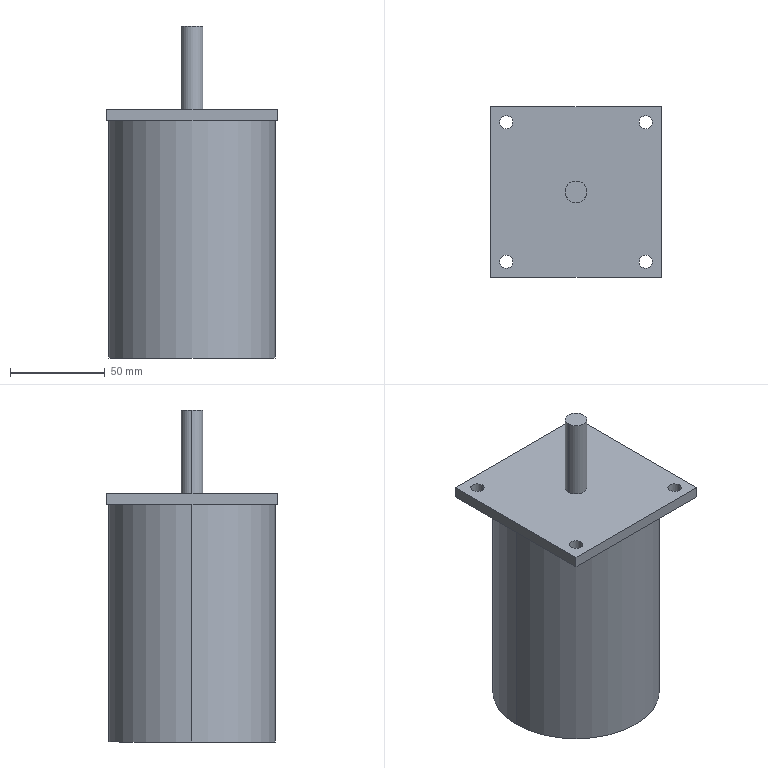Component | SolidWorks | Motor-1 | 1 solid | 20 faces | box 90 x 90 x 175 mm | volume 812512 mm3 | cylinder 12 | plane 8 | commonest cylinder face diameters 7 x8 11.5 x2 88 x2
build123d program:
from build123d import *

# Parameters (mm, degrees)
SKETCH1_W      = 90
SKETCH1_H      = 90
SKETCH1_R      = 3.5
EXTRUDE1_DEPTH = 6
SKETCH2_R      = 44
EXTRUDE2_DEPTH = 125
SKETCH3_R      = 5.75
EXTRUDE3_DEPTH = 44


with BuildPart() as part:
    # Sketch1 → Extrude1 (new body)
    with BuildSketch(Plane.XY):
        Rectangle(SKETCH1_W, SKETCH1_H)
        with Locations((-36.75, 36.75)):
            Circle(SKETCH1_R, mode=Mode.SUBTRACT)
        with Locations((36.75, 36.75)):
            Circle(SKETCH1_R, mode=Mode.SUBTRACT)
        with Locations((36.75, -36.75)):
            Circle(SKETCH1_R, mode=Mode.SUBTRACT)
        with Locations((-36.75, -36.75)):
            Circle(SKETCH1_R, mode=Mode.SUBTRACT)
    extrude(amount=EXTRUDE1_DEPTH)

    # Sketch2 → Extrude2 (add)
    with BuildSketch(Plane.XY.offset(6)):
        Circle(SKETCH2_R)
    extrude(amount=EXTRUDE2_DEPTH)

    # Sketch3 → Extrude3 (add)
    with BuildSketch(Plane(origin=(0, 0, 0), x_dir=(-1, 0, 0), z_dir=(0, 0, -1))):
        with Locations(Location((0, 0, 0), (0, 0, 180))):
            Circle(SKETCH3_R)
    extrude(amount=EXTRUDE3_DEPTH)


solid = part.part

# Placed as in the assembly
solid = solid.moved(Location((-160.944, 693.983, 237.789), (180, 0, 0)))
STEP:
#1=COLOUR_RGB('',0.7922,0.8196,0.9333);
#2=FILL_AREA_STYLE_COLOUR('',#1);
#3=FILL_AREA_STYLE('',(#2));
#4=SURFACE_STYLE_FILL_AREA(#3);
#5=SURFACE_SIDE_STYLE('',(#4));
#6=SURFACE_STYLE_USAGE(.BOTH.,#5);
#7=PRESENTATION_STYLE_ASSIGNMENT((#6));
#8=CARTESIAN_POINT('',(-6.11,27.322,11.094));
#9=VERTEX_POINT('',#8);
#10=CARTESIAN_POINT('',(-6.563,27.322,11.094));
#11=VERTEX_POINT('',#10);
#12=CARTESIAN_POINT('',(-6.336,27.322,11.094));
#13=DIRECTION('',(-0.,-0.,1.));
#14=DIRECTION('',(1.,0.,0.));
#15=AXIS2_PLACEMENT_3D('',#12,#13,#14);
#16=CIRCLE('',#15,0.2264);
#17=EDGE_CURVE('',#9,#11,#16,.T.);
#18=ORIENTED_EDGE('',*,*,#17,.F.);
#19=CARTESIAN_POINT('',(-6.11,27.322,9.362));
#20=VERTEX_POINT('',#19);
#21=CARTESIAN_POINT('',(-6.11,27.322,11.094));
#22=DIRECTION('',(0.,0.,-1.));
#23=VECTOR('',#22,39.37);
#24=LINE('',#21,#23);
#25=EDGE_CURVE('',#9,#20,#24,.T.);
#26=ORIENTED_EDGE('',*,*,#25,.T.);
#27=CARTESIAN_POINT('',(-6.563,27.322,9.362));
#28=VERTEX_POINT('',#27);
#29=CARTESIAN_POINT('',(-6.336,27.322,9.362));
#30=DIRECTION('',(-0.,-0.,1.));
#31=DIRECTION('',(-1.,0.,0.));
#32=AXIS2_PLACEMENT_3D('',#29,#30,#31);
#33=CIRCLE('',#32,0.2264);
#34=EDGE_CURVE('',#20,#28,#33,.T.);
#35=ORIENTED_EDGE('',*,*,#34,.T.);
#36=CARTESIAN_POINT('',(-6.563,27.322,11.094));
#37=DIRECTION('',(0.,0.,-1.));
#38=VECTOR('',#37,39.37);
#39=LINE('',#36,#38);
#40=EDGE_CURVE('',#11,#28,#39,.T.);
#41=ORIENTED_EDGE('',*,*,#40,.F.);
#42=EDGE_LOOP('',(#18,#26,#35,#41));
#43=FACE_OUTER_BOUND('',#42,.T.);
#44=CARTESIAN_POINT('',(-6.336,27.322,11.094));
#45=DIRECTION('',(0.,0.,-1.));
#46=DIRECTION('',(-1.,0.,0.));
#47=AXIS2_PLACEMENT_3D('',#44,#45,#46);
#48=CYLINDRICAL_SURFACE('',#47,0.2264);
#49=ADVANCED_FACE('',(#43),#48,.T.);
#50=CARTESIAN_POINT('',(-8.069,27.322,4.204));
#51=VERTEX_POINT('',#50);
#52=CARTESIAN_POINT('',(-4.604,27.322,4.204));
#53=VERTEX_POINT('',#52);
#54=CARTESIAN_POINT('',(-6.336,27.322,4.204));
#55=DIRECTION('',(0.,0.,-1.));
#56=DIRECTION('',(-1.,0.,0.));
#57=AXIS2_PLACEMENT_3D('',#54,#55,#56);
#58=CIRCLE('',#57,1.732);
#59=EDGE_CURVE('',#51,#53,#58,.T.);
#60=ORIENTED_EDGE('',*,*,#59,.F.);
#61=CARTESIAN_POINT('',(-8.069,27.322,9.126));
#62=VERTEX_POINT('',#61);
#63=CARTESIAN_POINT('',(-8.069,27.322,4.204));
#64=DIRECTION('',(-0.,-0.,1.));
#65=VECTOR('',#64,39.37);
#66=LINE('',#63,#65);
#67=EDGE_CURVE('',#51,#62,#66,.T.);
#68=ORIENTED_EDGE('',*,*,#67,.T.);
#69=CARTESIAN_POINT('',(-4.604,27.322,9.126));
#70=VERTEX_POINT('',#69);
#71=CARTESIAN_POINT('',(-6.336,27.322,9.126));
#72=DIRECTION('',(0.,0.,-1.));
#73=DIRECTION('',(-1.,0.,0.));
#74=AXIS2_PLACEMENT_3D('',#71,#72,#73);
#75=CIRCLE('',#74,1.732);
#76=EDGE_CURVE('',#62,#70,#75,.T.);
#77=ORIENTED_EDGE('',*,*,#76,.T.);
#78=CARTESIAN_POINT('',(-4.604,27.322,4.204));
#79=DIRECTION('',(-0.,-0.,1.));
#80=VECTOR('',#79,39.37);
#81=LINE('',#78,#80);
#82=EDGE_CURVE('',#53,#70,#81,.T.);
#83=ORIENTED_EDGE('',*,*,#82,.F.);
#84=EDGE_LOOP('',(#60,#68,#77,#83));
#85=FACE_OUTER_BOUND('',#84,.T.);
#86=CARTESIAN_POINT('',(-6.336,27.322,4.204));
#87=DIRECTION('',(-0.,-0.,1.));
#88=DIRECTION('',(1.,0.,0.));
#89=AXIS2_PLACEMENT_3D('',#86,#87,#88);
#90=CYLINDRICAL_SURFACE('',#89,1.732);
#91=ADVANCED_FACE('',(#85),#90,.T.);
#92=CARTESIAN_POINT('',(-4.752,25.875,9.126));
#93=VERTEX_POINT('',#92);
#94=CARTESIAN_POINT('',(-5.027,25.875,9.126));
#95=VERTEX_POINT('',#94);
#96=CARTESIAN_POINT('',(-4.89,25.875,9.126));
#97=DIRECTION('',(0.,0.,-1.));
#98=DIRECTION('',(-1.,0.,0.));
#99=AXIS2_PLACEMENT_3D('',#96,#97,#98);
#100=CIRCLE('',#99,0.1378);
#101=EDGE_CURVE('',#93,#95,#100,.T.);
#102=ORIENTED_EDGE('',*,*,#101,.T.);
#103=CARTESIAN_POINT('',(-5.027,25.875,9.362));
#104=VERTEX_POINT('',#103);
#105=CARTESIAN_POINT('',(-5.027,25.875,9.126));
#106=DIRECTION('',(-0.,-0.,1.));
#107=VECTOR('',#106,39.37);
#108=LINE('',#105,#107);
#109=EDGE_CURVE('',#95,#104,#108,.T.);
#110=ORIENTED_EDGE('',*,*,#109,.T.);
#111=CARTESIAN_POINT('',(-4.752,25.875,9.362));
#112=VERTEX_POINT('',#111);
#113=CARTESIAN_POINT('',(-4.89,25.875,9.362));
#114=DIRECTION('',(0.,0.,-1.));
#115=DIRECTION('',(-1.,0.,0.));
#116=AXIS2_PLACEMENT_3D('',#113,#114,#115);
#117=CIRCLE('',#116,0.1378);
#118=EDGE_CURVE('',#112,#104,#117,.T.);
#119=ORIENTED_EDGE('',*,*,#118,.F.);
#120=CARTESIAN_POINT('',(-4.752,25.875,9.126));
#121=DIRECTION('',(-0.,-0.,1.));
#122=VECTOR('',#121,39.37);
#123=LINE('',#120,#122);
#124=EDGE_CURVE('',#93,#112,#123,.T.);
#125=ORIENTED_EDGE('',*,*,#124,.F.);
#126=EDGE_LOOP('',(#102,#110,#119,#125));
#127=FACE_OUTER_BOUND('',#126,.T.);
#128=CARTESIAN_POINT('',(-4.89,25.875,9.126));
#129=DIRECTION('',(-0.,-0.,1.));
#130=DIRECTION('',(1.,0.,0.));
#131=AXIS2_PLACEMENT_3D('',#128,#129,#130);
#132=CYLINDRICAL_SURFACE('',#131,0.1378);
#133=ADVANCED_FACE('',(#127),#132,.F.);
#134=CARTESIAN_POINT('',(-7.645,25.875,9.126));
#135=VERTEX_POINT('',#134);
#136=CARTESIAN_POINT('',(-7.921,25.875,9.126));
#137=VERTEX_POINT('',#136);
#138=CARTESIAN_POINT('',(-7.783,25.875,9.126));
#139=DIRECTION('',(0.,0.,-1.));
#140=DIRECTION('',(-1.,0.,0.));
#141=AXIS2_PLACEMENT_3D('',#138,#139,#140);
#142=CIRCLE('',#141,0.1378);
#143=EDGE_CURVE('',#135,#137,#142,.T.);
#144=ORIENTED_EDGE('',*,*,#143,.T.);
#145=CARTESIAN_POINT('',(-7.921,25.875,9.362));
#146=VERTEX_POINT('',#145);
#147=CARTESIAN_POINT('',(-7.921,25.875,9.126));
#148=DIRECTION('',(-0.,-0.,1.));
#149=VECTOR('',#148,39.37);
#150=LINE('',#147,#149);
#151=EDGE_CURVE('',#137,#146,#150,.T.);
#152=ORIENTED_EDGE('',*,*,#151,.T.);
#153=CARTESIAN_POINT('',(-7.645,25.875,9.362));
#154=VERTEX_POINT('',#153);
#155=CARTESIAN_POINT('',(-7.783,25.875,9.362));
#156=DIRECTION('',(0.,0.,-1.));
#157=DIRECTION('',(-1.,0.,0.));
#158=AXIS2_PLACEMENT_3D('',#155,#156,#157);
#159=CIRCLE('',#158,0.1378);
#160=EDGE_CURVE('',#154,#146,#159,.T.);
#161=ORIENTED_EDGE('',*,*,#160,.F.);
#162=CARTESIAN_POINT('',(-7.645,25.875,9.126));
#163=DIRECTION('',(-0.,-0.,1.));
#164=VECTOR('',#163,39.37);
#165=LINE('',#162,#164);
#166=EDGE_CURVE('',#135,#154,#165,.T.);
#167=ORIENTED_EDGE('',*,*,#166,.F.);
#168=EDGE_LOOP('',(#144,#152,#161,#167));
#169=FACE_OUTER_BOUND('',#168,.T.);
#170=CARTESIAN_POINT('',(-7.783,25.875,9.126));
#171=DIRECTION('',(-0.,-0.,1.));
#172=DIRECTION('',(1.,0.,0.));
#173=AXIS2_PLACEMENT_3D('',#170,#171,#172);
#174=CYLINDRICAL_SURFACE('',#173,0.1378);
#175=ADVANCED_FACE('',(#169),#174,.F.);
#176=CARTESIAN_POINT('',(-7.645,28.769,9.126));
#177=VERTEX_POINT('',#176);
#178=CARTESIAN_POINT('',(-7.921,28.769,9.126));
#179=VERTEX_POINT('',#178);
#180=CARTESIAN_POINT('',(-7.783,28.769,9.126));
#181=DIRECTION('',(0.,0.,-1.));
#182=DIRECTION('',(-1.,0.,0.));
#183=AXIS2_PLACEMENT_3D('',#180,#181,#182);
#184=CIRCLE('',#183,0.1378);
#185=EDGE_CURVE('',#177,#179,#184,.T.);
#186=ORIENTED_EDGE('',*,*,#185,.T.);
#187=CARTESIAN_POINT('',(-7.921,28.769,9.362));
#188=VERTEX_POINT('',#187);
#189=CARTESIAN_POINT('',(-7.921,28.769,9.126));
#190=DIRECTION('',(-0.,-0.,1.));
#191=VECTOR('',#190,39.37);
#192=LINE('',#189,#191);
#193=EDGE_CURVE('',#179,#188,#192,.T.);
#194=ORIENTED_EDGE('',*,*,#193,.T.);
#195=CARTESIAN_POINT('',(-7.645,28.769,9.362));
#196=VERTEX_POINT('',#195);
#197=CARTESIAN_POINT('',(-7.783,28.769,9.362));
#198=DIRECTION('',(0.,0.,-1.));
#199=DIRECTION('',(-1.,0.,0.));
#200=AXIS2_PLACEMENT_3D('',#197,#198,#199);
#201=CIRCLE('',#200,0.1378);
#202=EDGE_CURVE('',#196,#188,#201,.T.);
#203=ORIENTED_EDGE('',*,*,#202,.F.);
#204=CARTESIAN_POINT('',(-7.645,28.769,9.126));
#205=DIRECTION('',(-0.,-0.,1.));
#206=VECTOR('',#205,39.37);
#207=LINE('',#204,#206);
#208=EDGE_CURVE('',#177,#196,#207,.T.);
#209=ORIENTED_EDGE('',*,*,#208,.F.);
#210=EDGE_LOOP('',(#186,#194,#203,#209));
#211=FACE_OUTER_BOUND('',#210,.T.);
#212=CARTESIAN_POINT('',(-7.783,28.769,9.126));
#213=DIRECTION('',(-0.,-0.,1.));
#214=DIRECTION('',(1.,0.,0.));
#215=AXIS2_PLACEMENT_3D('',#212,#213,#214);
#216=CYLINDRICAL_SURFACE('',#215,0.1378);
#217=ADVANCED_FACE('',(#211),#216,.F.);
#218=CARTESIAN_POINT('',(-4.752,28.769,9.126));
#219=VERTEX_POINT('',#218);
#220=CARTESIAN_POINT('',(-5.027,28.769,9.126));
#221=VERTEX_POINT('',#220);
#222=CARTESIAN_POINT('',(-4.89,28.769,9.126));
#223=DIRECTION('',(0.,0.,-1.));
#224=DIRECTION('',(-1.,0.,0.));
#225=AXIS2_PLACEMENT_3D('',#222,#223,#224);
#226=CIRCLE('',#225,0.1378);
#227=EDGE_CURVE('',#219,#221,#226,.T.);
#228=ORIENTED_EDGE('',*,*,#227,.T.);
#229=CARTESIAN_POINT('',(-5.027,28.769,9.362));
#230=VERTEX_POINT('',#229);
#231=CARTESIAN_POINT('',(-5.027,28.769,9.126));
#232=DIRECTION('',(-0.,-0.,1.));
#233=VECTOR('',#232,39.37);
#234=LINE('',#231,#233);
#235=EDGE_CURVE('',#221,#230,#234,.T.);
#236=ORIENTED_EDGE('',*,*,#235,.T.);
#237=CARTESIAN_POINT('',(-4.752,28.769,9.362));
#238=VERTEX_POINT('',#237);
#239=CARTESIAN_POINT('',(-4.89,28.769,9.362));
#240=DIRECTION('',(0.,0.,-1.));
#241=DIRECTION('',(-1.,0.,0.));
#242=AXIS2_PLACEMENT_3D('',#239,#240,#241);
#243=CIRCLE('',#242,0.1378);
#244=EDGE_CURVE('',#238,#230,#243,.T.);
#245=ORIENTED_EDGE('',*,*,#244,.F.);
#246=CARTESIAN_POINT('',(-4.752,28.769,9.126));
#247=DIRECTION('',(-0.,-0.,1.));
#248=VECTOR('',#247,39.37);
#249=LINE('',#246,#248);
#250=EDGE_CURVE('',#219,#238,#249,.T.);
#251=ORIENTED_EDGE('',*,*,#250,.F.);
#252=EDGE_LOOP('',(#228,#236,#245,#251));
#253=FACE_OUTER_BOUND('',#252,.T.);
#254=CARTESIAN_POINT('',(-4.89,28.769,9.126));
#255=DIRECTION('',(-0.,-0.,1.));
#256=DIRECTION('',(1.,0.,0.));
#257=AXIS2_PLACEMENT_3D('',#254,#255,#256);
#258=CYLINDRICAL_SURFACE('',#257,0.1378);
#259=ADVANCED_FACE('',(#253),#258,.F.);
#260=CARTESIAN_POINT('',(-4.565,29.094,9.362));
#261=VERTEX_POINT('',#260);
#262=CARTESIAN_POINT('',(-4.565,25.551,9.362));
#263=VERTEX_POINT('',#262);
#264=CARTESIAN_POINT('',(-4.565,29.094,9.362));
#265=DIRECTION('',(-0.,-1.,-0.));
#266=VECTOR('',#265,39.37);
#267=LINE('',#264,#266);
#268=EDGE_CURVE('',#261,#263,#267,.T.);
#269=ORIENTED_EDGE('',*,*,#268,.F.);
#270=CARTESIAN_POINT('',(-8.108,29.094,9.362));
#271=VERTEX_POINT('',#270);
#272=CARTESIAN_POINT('',(-4.565,29.094,9.362));
#273=DIRECTION('',(1.,-0.,0.));
#274=VECTOR('',#273,39.37);
#275=LINE('',#272,#274);
#276=EDGE_CURVE('',#271,#261,#275,.T.);
#277=ORIENTED_EDGE('',*,*,#276,.F.);
#278=CARTESIAN_POINT('',(-8.108,25.551,9.362));
#279=VERTEX_POINT('',#278);
#280=CARTESIAN_POINT('',(-8.108,29.094,9.362));
#281=DIRECTION('',(0.,1.,0.));
#282=VECTOR('',#281,39.37);
#283=LINE('',#280,#282);
#284=EDGE_CURVE('',#279,#271,#283,.T.);
#285=ORIENTED_EDGE('',*,*,#284,.F.);
#286=CARTESIAN_POINT('',(-4.565,25.551,9.362));
#287=DIRECTION('',(-1.,0.,-0.));
#288=VECTOR('',#287,39.37);
#289=LINE('',#286,#288);
#290=EDGE_CURVE('',#263,#279,#289,.T.);
#291=ORIENTED_EDGE('',*,*,#290,.F.);
#292=EDGE_LOOP('',(#269,#277,#285,#291));
#293=FACE_OUTER_BOUND('',#292,.T.);
#294=ORIENTED_EDGE('',*,*,#244,.T.);
#295=CARTESIAN_POINT('',(-4.89,28.769,9.362));
#296=DIRECTION('',(0.,0.,-1.));
#297=DIRECTION('',(-1.,0.,0.));
#298=AXIS2_PLACEMENT_3D('',#295,#296,#297);
#299=CIRCLE('',#298,0.1378);
#300=EDGE_CURVE('',#230,#238,#299,.T.);
#301=ORIENTED_EDGE('',*,*,#300,.T.);
#302=EDGE_LOOP('',(#294,#301));
#303=FACE_BOUND('',#302,.T.);
#304=ORIENTED_EDGE('',*,*,#202,.T.);
#305=CARTESIAN_POINT('',(-7.783,28.769,9.362));
#306=DIRECTION('',(0.,0.,-1.));
#307=DIRECTION('',(-1.,0.,0.));
#308=AXIS2_PLACEMENT_3D('',#305,#306,#307);
#309=CIRCLE('',#308,0.1378);
#310=EDGE_CURVE('',#188,#196,#309,.T.);
#311=ORIENTED_EDGE('',*,*,#310,.T.);
#312=EDGE_LOOP('',(#304,#311));
#313=FACE_BOUND('',#312,.T.);
#314=ORIENTED_EDGE('',*,*,#160,.T.);
#315=CARTESIAN_POINT('',(-7.783,25.875,9.362));
#316=DIRECTION('',(0.,0.,-1.));
#317=DIRECTION('',(-1.,0.,0.));
#318=AXIS2_PLACEMENT_3D('',#315,#316,#317);
#319=CIRCLE('',#318,0.1378);
#320=EDGE_CURVE('',#146,#154,#319,.T.);
#321=ORIENTED_EDGE('',*,*,#320,.T.);
#322=EDGE_LOOP('',(#314,#321));
#323=FACE_BOUND('',#322,.T.);
#324=ORIENTED_EDGE('',*,*,#118,.T.);
#325=CARTESIAN_POINT('',(-4.89,25.875,9.362));
#326=DIRECTION('',(0.,0.,-1.));
#327=DIRECTION('',(-1.,0.,0.));
#328=AXIS2_PLACEMENT_3D('',#325,#326,#327);
#329=CIRCLE('',#328,0.1378);
#330=EDGE_CURVE('',#104,#112,#329,.T.);
#331=ORIENTED_EDGE('',*,*,#330,.T.);
#332=EDGE_LOOP('',(#324,#331));
#333=FACE_BOUND('',#332,.T.);
#334=CARTESIAN_POINT('',(-6.336,27.322,9.362));
#335=DIRECTION('',(-0.,-0.,1.));
#336=DIRECTION('',(-1.,0.,0.));
#337=AXIS2_PLACEMENT_3D('',#334,#335,#336);
#338=CIRCLE('',#337,0.2264);
#339=EDGE_CURVE('',#28,#20,#338,.T.);
#340=ORIENTED_EDGE('',*,*,#339,.F.);
#341=ORIENTED_EDGE('',*,*,#34,.F.);
#342=EDGE_LOOP('',(#340,#341));
#343=FACE_BOUND('',#342,.T.);
#344=CARTESIAN_POINT('',(-4.565,25.551,9.362));
#345=DIRECTION('',(0.,0.,-1.));
#346=DIRECTION('',(-1.,0.,-0.));
#347=AXIS2_PLACEMENT_3D('',#344,#345,#346);
#348=PLANE('',#347);
#349=ADVANCED_FACE('',(#293,#303,#313,#323,#333,#343),#348,.F.);
#350=ORIENTED_EDGE('',*,*,#101,.F.);
#351=CARTESIAN_POINT('',(-4.89,25.875,9.126));
#352=DIRECTION('',(0.,0.,-1.));
#353=DIRECTION('',(-1.,0.,0.));
#354=AXIS2_PLACEMENT_3D('',#351,#352,#353);
#355=CIRCLE('',#354,0.1378);
#356=EDGE_CURVE('',#95,#93,#355,.T.);
#357=ORIENTED_EDGE('',*,*,#356,.F.);
#358=EDGE_LOOP('',(#350,#357));
#359=FACE_BOUND('',#358,.T.);
#360=ORIENTED_EDGE('',*,*,#185,.F.);
#361=CARTESIAN_POINT('',(-7.783,28.769,9.126));
#362=DIRECTION('',(0.,0.,-1.));
#363=DIRECTION('',(-1.,0.,0.));
#364=AXIS2_PLACEMENT_3D('',#361,#362,#363);
#365=CIRCLE('',#364,0.1378);
#366=EDGE_CURVE('',#179,#177,#365,.T.);
#367=ORIENTED_EDGE('',*,*,#366,.F.);
#368=EDGE_LOOP('',(#360,#367));
#369=FACE_BOUND('',#368,.T.);
#370=CARTESIAN_POINT('',(-4.565,29.094,9.126));
#371=VERTEX_POINT('',#370);
#372=CARTESIAN_POINT('',(-4.565,25.551,9.126));
#373=VERTEX_POINT('',#372);
#374=CARTESIAN_POINT('',(-4.565,29.094,9.126));
#375=DIRECTION('',(-0.,-1.,-0.));
#376=VECTOR('',#375,39.37);
#377=LINE('',#374,#376);
#378=EDGE_CURVE('',#371,#373,#377,.T.);
#379=ORIENTED_EDGE('',*,*,#378,.T.);
#380=CARTESIAN_POINT('',(-8.108,25.551,9.126));
#381=VERTEX_POINT('',#380);
#382=CARTESIAN_POINT('',(-4.565,25.551,9.126));
#383=DIRECTION('',(-1.,0.,-0.));
#384=VECTOR('',#383,39.37);
#385=LINE('',#382,#384);
#386=EDGE_CURVE('',#373,#381,#385,.T.);
#387=ORIENTED_EDGE('',*,*,#386,.T.);
#388=CARTESIAN_POINT('',(-8.108,29.094,9.126));
#389=VERTEX_POINT('',#388);
#390=CARTESIAN_POINT('',(-8.108,29.094,9.126));
#391=DIRECTION('',(0.,1.,0.));
#392=VECTOR('',#391,39.37);
#393=LINE('',#390,#392);
#394=EDGE_CURVE('',#381,#389,#393,.T.);
#395=ORIENTED_EDGE('',*,*,#394,.T.);
#396=CARTESIAN_POINT('',(-4.565,29.094,9.126));
#397=DIRECTION('',(1.,-0.,0.));
#398=VECTOR('',#397,39.37);
#399=LINE('',#396,#398);
#400=EDGE_CURVE('',#389,#371,#399,.T.);
#401=ORIENTED_EDGE('',*,*,#400,.T.);
#402=EDGE_LOOP('',(#379,#387,#395,#401));
#403=FACE_OUTER_BOUND('',#402,.T.);
#404=ORIENTED_EDGE('',*,*,#227,.F.);
#405=CARTESIAN_POINT('',(-4.89,28.769,9.126));
#406=DIRECTION('',(0.,0.,-1.));
#407=DIRECTION('',(-1.,0.,0.));
#408=AXIS2_PLACEMENT_3D('',#405,#406,#407);
#409=CIRCLE('',#408,0.1378);
#410=EDGE_CURVE('',#221,#219,#409,.T.);
#411=ORIENTED_EDGE('',*,*,#410,.F.);
#412=EDGE_LOOP('',(#404,#411));
#413=FACE_BOUND('',#412,.T.);
#414=ORIENTED_EDGE('',*,*,#143,.F.);
#415=CARTESIAN_POINT('',(-7.783,25.875,9.126));
#416=DIRECTION('',(0.,0.,-1.));
#417=DIRECTION('',(-1.,0.,0.));
#418=AXIS2_PLACEMENT_3D('',#415,#416,#417);
#419=CIRCLE('',#418,0.1378);
#420=EDGE_CURVE('',#137,#135,#419,.T.);
#421=ORIENTED_EDGE('',*,*,#420,.F.);
#422=EDGE_LOOP('',(#414,#421));
#423=FACE_BOUND('',#422,.T.);
#424=CARTESIAN_POINT('',(-6.336,27.322,9.126));
#425=DIRECTION('',(0.,0.,-1.));
#426=DIRECTION('',(-1.,0.,0.));
#427=AXIS2_PLACEMENT_3D('',#424,#425,#426);
#428=CIRCLE('',#427,1.732);
#429=EDGE_CURVE('',#70,#62,#428,.T.);
#430=ORIENTED_EDGE('',*,*,#429,.F.);
#431=ORIENTED_EDGE('',*,*,#76,.F.);
#432=EDGE_LOOP('',(#430,#431));
#433=FACE_BOUND('',#432,.T.);
#434=CARTESIAN_POINT('',(-4.565,25.551,9.126));
#435=DIRECTION('',(0.,0.,-1.));
#436=DIRECTION('',(-1.,0.,-0.));
#437=AXIS2_PLACEMENT_3D('',#434,#435,#436);
#438=PLANE('',#437);
#439=ADVANCED_FACE('',(#359,#369,#403,#413,#423,#433),#438,.T.);
#440=ORIENTED_EDGE('',*,*,#268,.T.);
#441=CARTESIAN_POINT('',(-4.565,25.551,9.126));
#442=DIRECTION('',(-0.,-0.,1.));
#443=VECTOR('',#442,39.37);
#444=LINE('',#441,#443);
#445=EDGE_CURVE('',#373,#263,#444,.T.);
#446=ORIENTED_EDGE('',*,*,#445,.F.);
#447=ORIENTED_EDGE('',*,*,#378,.F.);
#448=CARTESIAN_POINT('',(-4.565,29.094,9.126));
#449=DIRECTION('',(-0.,-0.,1.));
#450=VECTOR('',#449,39.37);
#451=LINE('',#448,#450);
#452=EDGE_CURVE('',#371,#261,#451,.T.);
#453=ORIENTED_EDGE('',*,*,#452,.T.);
#454=EDGE_LOOP('',(#440,#446,#447,#453));
#455=FACE_OUTER_BOUND('',#454,.T.);
#456=CARTESIAN_POINT('',(-4.565,29.094,9.126));
#457=DIRECTION('',(-1.,0.,-0.));
#458=DIRECTION('',(0.,1.,0.));
#459=AXIS2_PLACEMENT_3D('',#456,#457,#458);
#460=PLANE('',#459);
#461=ADVANCED_FACE('',(#455),#460,.F.);
#462=ORIENTED_EDGE('',*,*,#290,.T.);
#463=CARTESIAN_POINT('',(-8.108,25.551,9.126));
#464=DIRECTION('',(-0.,-0.,1.));
#465=VECTOR('',#464,39.37);
#466=LINE('',#463,#465);
#467=EDGE_CURVE('',#381,#279,#466,.T.);
#468=ORIENTED_EDGE('',*,*,#467,.F.);
#469=ORIENTED_EDGE('',*,*,#386,.F.);
#470=ORIENTED_EDGE('',*,*,#445,.T.);
#471=EDGE_LOOP('',(#462,#468,#469,#470));
#472=FACE_OUTER_BOUND('',#471,.T.);
#473=CARTESIAN_POINT('',(-4.565,25.551,9.126));
#474=DIRECTION('',(0.,1.,0.));
#475=DIRECTION('',(0.,0.,-1.));
#476=AXIS2_PLACEMENT_3D('',#473,#474,#475);
#477=PLANE('',#476);
#478=ADVANCED_FACE('',(#472),#477,.F.);
#479=ORIENTED_EDGE('',*,*,#284,.T.);
#480=CARTESIAN_POINT('',(-8.108,29.094,9.126));
#481=DIRECTION('',(-0.,-0.,1.));
#482=VECTOR('',#481,39.37);
#483=LINE('',#480,#482);
#484=EDGE_CURVE('',#389,#271,#483,.T.);
#485=ORIENTED_EDGE('',*,*,#484,.F.);
#486=ORIENTED_EDGE('',*,*,#394,.F.);
#487=ORIENTED_EDGE('',*,*,#467,.T.);
#488=EDGE_LOOP('',(#479,#485,#486,#487));
#489=FACE_OUTER_BOUND('',#488,.T.);
#490=CARTESIAN_POINT('',(-8.108,29.094,9.126));
#491=DIRECTION('',(1.,-0.,0.));
#492=DIRECTION('',(-0.,-1.,-0.));
#493=AXIS2_PLACEMENT_3D('',#490,#491,#492);
#494=PLANE('',#493);
#495=ADVANCED_FACE('',(#489),#494,.F.);
#496=ORIENTED_EDGE('',*,*,#276,.T.);
#497=ORIENTED_EDGE('',*,*,#452,.F.);
#498=ORIENTED_EDGE('',*,*,#400,.F.);
#499=ORIENTED_EDGE('',*,*,#484,.T.);
#500=EDGE_LOOP('',(#496,#497,#498,#499));
#501=FACE_OUTER_BOUND('',#500,.T.);
#502=CARTESIAN_POINT('',(-4.565,29.094,9.126));
#503=DIRECTION('',(-0.,-1.,-0.));
#504=DIRECTION('',(-0.,-0.,1.));
#505=AXIS2_PLACEMENT_3D('',#502,#503,#504);
#506=PLANE('',#505);
#507=ADVANCED_FACE('',(#501),#506,.F.);
#508=ORIENTED_EDGE('',*,*,#235,.F.);
#509=ORIENTED_EDGE('',*,*,#410,.T.);
#510=ORIENTED_EDGE('',*,*,#250,.T.);
#511=ORIENTED_EDGE('',*,*,#300,.F.);
#512=EDGE_LOOP('',(#508,#509,#510,#511));
#513=FACE_OUTER_BOUND('',#512,.T.);
#514=CARTESIAN_POINT('',(-4.89,28.769,9.126));
#515=DIRECTION('',(-0.,-0.,1.));
#516=DIRECTION('',(1.,0.,0.));
#517=AXIS2_PLACEMENT_3D('',#514,#515,#516);
#518=CYLINDRICAL_SURFACE('',#517,0.1378);
#519=ADVANCED_FACE('',(#513),#518,.F.);
#520=ORIENTED_EDGE('',*,*,#193,.F.);
#521=ORIENTED_EDGE('',*,*,#366,.T.);
#522=ORIENTED_EDGE('',*,*,#208,.T.);
#523=ORIENTED_EDGE('',*,*,#310,.F.);
#524=EDGE_LOOP('',(#520,#521,#522,#523));
#525=FACE_OUTER_BOUND('',#524,.T.);
#526=CARTESIAN_POINT('',(-7.783,28.769,9.126));
#527=DIRECTION('',(-0.,-0.,1.));
#528=DIRECTION('',(1.,0.,0.));
#529=AXIS2_PLACEMENT_3D('',#526,#527,#528);
#530=CYLINDRICAL_SURFACE('',#529,0.1378);
#531=ADVANCED_FACE('',(#525),#530,.F.);
#532=ORIENTED_EDGE('',*,*,#151,.F.);
#533=ORIENTED_EDGE('',*,*,#420,.T.);
#534=ORIENTED_EDGE('',*,*,#166,.T.);
#535=ORIENTED_EDGE('',*,*,#320,.F.);
#536=EDGE_LOOP('',(#532,#533,#534,#535));
#537=FACE_OUTER_BOUND('',#536,.T.);
#538=CARTESIAN_POINT('',(-7.783,25.875,9.126));
#539=DIRECTION('',(-0.,-0.,1.));
#540=DIRECTION('',(1.,0.,0.));
#541=AXIS2_PLACEMENT_3D('',#538,#539,#540);
#542=CYLINDRICAL_SURFACE('',#541,0.1378);
#543=ADVANCED_FACE('',(#537),#542,.F.);
#544=ORIENTED_EDGE('',*,*,#109,.F.);
#545=ORIENTED_EDGE('',*,*,#356,.T.);
#546=ORIENTED_EDGE('',*,*,#124,.T.);
#547=ORIENTED_EDGE('',*,*,#330,.F.);
#548=EDGE_LOOP('',(#544,#545,#546,#547));
#549=FACE_OUTER_BOUND('',#548,.T.);
#550=CARTESIAN_POINT('',(-4.89,25.875,9.126));
#551=DIRECTION('',(-0.,-0.,1.));
#552=DIRECTION('',(1.,0.,0.));
#553=AXIS2_PLACEMENT_3D('',#550,#551,#552);
#554=CYLINDRICAL_SURFACE('',#553,0.1378);
#555=ADVANCED_FACE('',(#549),#554,.F.);
#556=ORIENTED_EDGE('',*,*,#67,.F.);
#557=CARTESIAN_POINT('',(-6.336,27.322,4.204));
#558=DIRECTION('',(0.,0.,-1.));
#559=DIRECTION('',(-1.,0.,0.));
#560=AXIS2_PLACEMENT_3D('',#557,#558,#559);
#561=CIRCLE('',#560,1.732);
#562=EDGE_CURVE('',#53,#51,#561,.T.);
#563=ORIENTED_EDGE('',*,*,#562,.F.);
#564=ORIENTED_EDGE('',*,*,#82,.T.);
#565=ORIENTED_EDGE('',*,*,#429,.T.);
#566=EDGE_LOOP('',(#556,#563,#564,#565));
#567=FACE_OUTER_BOUND('',#566,.T.);
#568=CARTESIAN_POINT('',(-6.336,27.322,4.204));
#569=DIRECTION('',(-0.,-0.,1.));
#570=DIRECTION('',(1.,0.,0.));
#571=AXIS2_PLACEMENT_3D('',#568,#569,#570);
#572=CYLINDRICAL_SURFACE('',#571,1.732);
#573=ADVANCED_FACE('',(#567),#572,.T.);
#574=ORIENTED_EDGE('',*,*,#562,.T.);
#575=ORIENTED_EDGE('',*,*,#59,.T.);
#576=EDGE_LOOP('',(#574,#575));
#577=FACE_OUTER_BOUND('',#576,.T.);
#578=CARTESIAN_POINT('',(-6.336,27.322,4.204));
#579=DIRECTION('',(0.,0.,-1.));
#580=DIRECTION('',(-1.,0.,-0.));
#581=AXIS2_PLACEMENT_3D('',#578,#579,#580);
#582=PLANE('',#581);
#583=ADVANCED_FACE('',(#577),#582,.T.);
#584=ORIENTED_EDGE('',*,*,#25,.F.);
#585=CARTESIAN_POINT('',(-6.336,27.322,11.094));
#586=DIRECTION('',(-0.,-0.,1.));
#587=DIRECTION('',(1.,0.,0.));
#588=AXIS2_PLACEMENT_3D('',#585,#586,#587);
#589=CIRCLE('',#588,0.2264);
#590=EDGE_CURVE('',#11,#9,#589,.T.);
#591=ORIENTED_EDGE('',*,*,#590,.F.);
#592=ORIENTED_EDGE('',*,*,#40,.T.);
#593=ORIENTED_EDGE('',*,*,#339,.T.);
#594=EDGE_LOOP('',(#584,#591,#592,#593));
#595=FACE_OUTER_BOUND('',#594,.T.);
#596=CARTESIAN_POINT('',(-6.336,27.322,11.094));
#597=DIRECTION('',(0.,0.,-1.));
#598=DIRECTION('',(-1.,0.,0.));
#599=AXIS2_PLACEMENT_3D('',#596,#597,#598);
#600=CYLINDRICAL_SURFACE('',#599,0.2264);
#601=ADVANCED_FACE('',(#595),#600,.T.);
#602=ORIENTED_EDGE('',*,*,#590,.T.);
#603=ORIENTED_EDGE('',*,*,#17,.T.);
#604=EDGE_LOOP('',(#602,#603));
#605=FACE_OUTER_BOUND('',#604,.T.);
#606=CARTESIAN_POINT('',(-6.336,27.322,11.094));
#607=DIRECTION('',(-0.,-0.,1.));
#608=DIRECTION('',(1.,-0.,0.));
#609=AXIS2_PLACEMENT_3D('',#606,#607,#608);
#610=PLANE('',#609);
#611=ADVANCED_FACE('',(#605),#610,.T.);
#612=CLOSED_SHELL('',(#49,#91,#133,#175,#217,#259,#349,#439,#461,#478,#495,#507,#519,#531,#543,#555,#573,#583,#601,#611));
#613=MANIFOLD_SOLID_BREP('',#612);
#614=STYLED_ITEM('',(#7),#613);
#615=(LENGTH_UNIT()NAMED_UNIT(*)SI_UNIT($,.METRE.));
#616=LENGTH_MEASURE_WITH_UNIT(LENGTH_MEASURE(0.0254),#615);
#617=DIMENSIONAL_EXPONENTS(1.,0.,0.,0.,0.,0.,0.);
#618=(CONVERSION_BASED_UNIT('',#616)LENGTH_UNIT()NAMED_UNIT(#617));
#619=UNCERTAINTY_MEASURE_WITH_UNIT(LENGTH_MEASURE(0.00001),#618,'','');
#620=(NAMED_UNIT(*)PLANE_ANGLE_UNIT()SI_UNIT($,.RADIAN.));
#621=(NAMED_UNIT(*)SI_UNIT($,.STERADIAN.)SOLID_ANGLE_UNIT());
#622=(GEOMETRIC_REPRESENTATION_CONTEXT(3)GLOBAL_UNCERTAINTY_ASSIGNED_CONTEXT((#619))GLOBAL_UNIT_ASSIGNED_CONTEXT((#618,#620,#621))REPRESENTATION_CONTEXT('',''));
#623=MECHANICAL_DESIGN_GEOMETRIC_PRESENTATION_REPRESENTATION('',(#614),#622);
#624=CARTESIAN_POINT('',(0.,0.,0.));
#625=DIRECTION('',(0.,0.,1.));
#626=DIRECTION('',(1.,0.,0.));
#627=AXIS2_PLACEMENT_3D('',#624,#625,#626);
#628=(LENGTH_UNIT()NAMED_UNIT(*)SI_UNIT($,.METRE.));
#629=LENGTH_MEASURE_WITH_UNIT(LENGTH_MEASURE(0.0254),#628);
#630=DIMENSIONAL_EXPONENTS(1.,0.,0.,0.,0.,0.,0.);
#631=(CONVERSION_BASED_UNIT('',#629)LENGTH_UNIT()NAMED_UNIT(#630));
#632=UNCERTAINTY_MEASURE_WITH_UNIT(LENGTH_MEASURE(0.00001),#631,'','');
#633=(NAMED_UNIT(*)PLANE_ANGLE_UNIT()SI_UNIT($,.RADIAN.));
#634=(NAMED_UNIT(*)SI_UNIT($,.STERADIAN.)SOLID_ANGLE_UNIT());
#635=(GEOMETRIC_REPRESENTATION_CONTEXT(3)GLOBAL_UNCERTAINTY_ASSIGNED_CONTEXT((#632))GLOBAL_UNIT_ASSIGNED_CONTEXT((#631,#633,#634))REPRESENTATION_CONTEXT('',''));
#636=ADVANCED_BREP_SHAPE_REPRESENTATION('',(#613,#627),#635);
#637=PRESENTATION_LAYER_ASSIGNMENT('','',(#614));